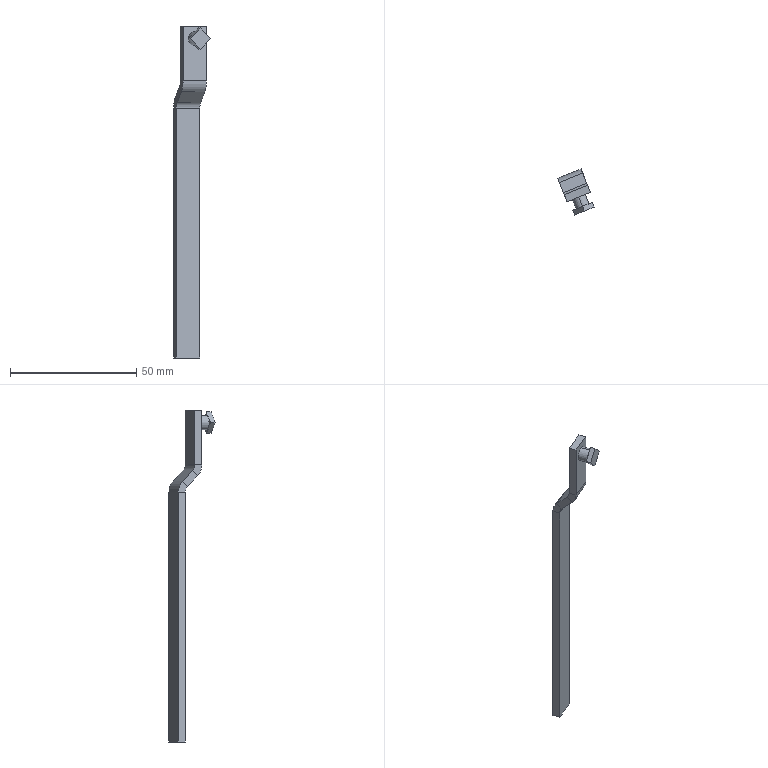Component | SolidWorks | RightDoorAssembly-1_LinkRodLock-1_Lock-1_UpperRod-1 | 1 solid | 30 faces | box 14.56 x 18.3 x 131.5 mm | volume 4187 mm3 | plane 24 | cylinder 6 | commonest cylinder face diameters 5.5 x2 6 x2 12 x2
STEP:
#1=COLOUR_RGB('',0.7922,0.8196,0.9333);
#2=FILL_AREA_STYLE_COLOUR('',#1);
#3=FILL_AREA_STYLE('',(#2));
#4=SURFACE_STYLE_FILL_AREA(#3);
#5=SURFACE_SIDE_STYLE('',(#4));
#6=SURFACE_STYLE_USAGE(.BOTH.,#5);
#7=PRESENTATION_STYLE_ASSIGNMENT((#6));
#8=CARTESIAN_POINT('',(-12.815,15.759,40.707));
#9=VERTEX_POINT('',#8);
#10=CARTESIAN_POINT('',(-12.815,15.759,40.49));
#11=VERTEX_POINT('',#10);
#12=CARTESIAN_POINT('',(-12.815,15.759,40.598));
#13=DIRECTION('',(0.3744,-0.9273,0.));
#14=DIRECTION('',(0.,0.,1.));
#15=AXIS2_PLACEMENT_3D('',#12,#13,#14);
#16=CIRCLE('',#15,0.1083);
#17=EDGE_CURVE('',#9,#11,#16,.T.);
#18=ORIENTED_EDGE('',*,*,#17,.F.);
#19=CARTESIAN_POINT('',(-12.874,15.905,40.707));
#20=VERTEX_POINT('',#19);
#21=CARTESIAN_POINT('',(-12.815,15.759,40.707));
#22=DIRECTION('',(-0.3744,0.9273,-0.));
#23=VECTOR('',#22,39.37);
#24=LINE('',#21,#23);
#25=EDGE_CURVE('',#9,#20,#24,.T.);
#26=ORIENTED_EDGE('',*,*,#25,.T.);
#27=CARTESIAN_POINT('',(-12.874,15.905,40.49));
#28=VERTEX_POINT('',#27);
#29=CARTESIAN_POINT('',(-12.874,15.905,40.598));
#30=DIRECTION('',(0.3744,-0.9273,0.));
#31=DIRECTION('',(0.,0.,-1.));
#32=AXIS2_PLACEMENT_3D('',#29,#30,#31);
#33=CIRCLE('',#32,0.1083);
#34=EDGE_CURVE('',#20,#28,#33,.T.);
#35=ORIENTED_EDGE('',*,*,#34,.T.);
#36=CARTESIAN_POINT('',(-12.815,15.759,40.49));
#37=DIRECTION('',(-0.3744,0.9273,-0.));
#38=VECTOR('',#37,39.37);
#39=LINE('',#36,#38);
#40=EDGE_CURVE('',#11,#28,#39,.T.);
#41=ORIENTED_EDGE('',*,*,#40,.F.);
#42=EDGE_LOOP('',(#18,#26,#35,#41));
#43=FACE_OUTER_BOUND('',#42,.T.);
#44=CARTESIAN_POINT('',(-12.815,15.759,40.598));
#45=DIRECTION('',(-0.3744,0.9273,-0.));
#46=DIRECTION('',(0.,0.,-1.));
#47=AXIS2_PLACEMENT_3D('',#44,#45,#46);
#48=CYLINDRICAL_SURFACE('',#47,0.1083);
#49=ADVANCED_FACE('',(#43),#48,.T.);
#50=CARTESIAN_POINT('',(-12.691,15.979,39.939));
#51=VERTEX_POINT('',#50);
#52=CARTESIAN_POINT('',(-12.691,15.979,40.795));
#53=VERTEX_POINT('',#52);
#54=CARTESIAN_POINT('',(-12.691,15.979,39.939));
#55=DIRECTION('',(-0.,0.,1.));
#56=VECTOR('',#55,39.37);
#57=LINE('',#54,#56);
#58=EDGE_CURVE('',#51,#53,#57,.T.);
#59=ORIENTED_EDGE('',*,*,#58,.T.);
#60=CARTESIAN_POINT('',(-13.056,15.832,40.795));
#61=VERTEX_POINT('',#60);
#62=CARTESIAN_POINT('',(-13.056,15.832,40.795));
#63=DIRECTION('',(0.9273,0.3744,0.));
#64=VECTOR('',#63,39.37);
#65=LINE('',#62,#64);
#66=EDGE_CURVE('',#61,#53,#65,.T.);
#67=ORIENTED_EDGE('',*,*,#66,.F.);
#68=CARTESIAN_POINT('',(-13.056,15.832,39.939));
#69=VERTEX_POINT('',#68);
#70=CARTESIAN_POINT('',(-13.056,15.832,39.939));
#71=DIRECTION('',(-0.,0.,1.));
#72=VECTOR('',#71,39.37);
#73=LINE('',#70,#72);
#74=EDGE_CURVE('',#69,#61,#73,.T.);
#75=ORIENTED_EDGE('',*,*,#74,.F.);
#76=CARTESIAN_POINT('',(-13.056,15.832,39.939));
#77=DIRECTION('',(0.9273,0.3744,0.));
#78=VECTOR('',#77,39.37);
#79=LINE('',#76,#78);
#80=EDGE_CURVE('',#69,#51,#79,.T.);
#81=ORIENTED_EDGE('',*,*,#80,.T.);
#82=EDGE_LOOP('',(#59,#67,#75,#81));
#83=FACE_OUTER_BOUND('',#82,.T.);
#84=CARTESIAN_POINT('',(-12.874,15.905,40.598));
#85=DIRECTION('',(0.3744,-0.9273,0.));
#86=DIRECTION('',(0.,0.,-1.));
#87=AXIS2_PLACEMENT_3D('',#84,#85,#86);
#88=CIRCLE('',#87,0.1083);
#89=EDGE_CURVE('',#28,#20,#88,.T.);
#90=ORIENTED_EDGE('',*,*,#89,.F.);
#91=ORIENTED_EDGE('',*,*,#34,.F.);
#92=EDGE_LOOP('',(#90,#91));
#93=FACE_BOUND('',#92,.T.);
#94=CARTESIAN_POINT('',(-13.056,15.832,39.939));
#95=DIRECTION('',(-0.3744,0.9273,-0.));
#96=DIRECTION('',(0.,-0.,-1.));
#97=AXIS2_PLACEMENT_3D('',#94,#95,#96);
#98=PLANE('',#97);
#99=ADVANCED_FACE('',(#83,#93),#98,.F.);
#100=CARTESIAN_POINT('',(-13.178,16.133,39.683));
#101=VERTEX_POINT('',#100);
#102=CARTESIAN_POINT('',(-13.146,16.055,39.6));
#103=VERTEX_POINT('',#102);
#104=CARTESIAN_POINT('',(-13.178,16.133,39.683));
#105=DIRECTION('',(0.2647,-0.6557,-0.7071));
#106=VECTOR('',#105,39.37);
#107=LINE('',#104,#106);
#108=EDGE_CURVE('',#101,#103,#107,.T.);
#109=ORIENTED_EDGE('',*,*,#108,.F.);
#110=CARTESIAN_POINT('',(-13.204,16.197,39.516));
#111=VERTEX_POINT('',#110);
#112=CARTESIAN_POINT('',(-13.115,15.978,39.516));
#113=DIRECTION('',(0.9273,0.3744,0.));
#114=DIRECTION('',(0.3744,-0.9273,0.));
#115=AXIS2_PLACEMENT_3D('',#112,#113,#114);
#116=CIRCLE('',#115,0.2362);
#117=EDGE_CURVE('',#111,#101,#116,.T.);
#118=ORIENTED_EDGE('',*,*,#117,.F.);
#119=CARTESIAN_POINT('',(-13.159,16.087,39.516));
#120=VERTEX_POINT('',#119);
#121=CARTESIAN_POINT('',(-13.159,16.087,39.516));
#122=DIRECTION('',(-0.3744,0.9273,-0.));
#123=VECTOR('',#122,39.37);
#124=LINE('',#121,#123);
#125=EDGE_CURVE('',#120,#111,#124,.T.);
#126=ORIENTED_EDGE('',*,*,#125,.F.);
#127=CARTESIAN_POINT('',(-13.115,15.978,39.516));
#128=DIRECTION('',(0.9273,0.3744,0.));
#129=DIRECTION('',(0.3744,-0.9273,-0.));
#130=AXIS2_PLACEMENT_3D('',#127,#128,#129);
#131=CIRCLE('',#130,0.1181);
#132=EDGE_CURVE('',#120,#103,#131,.T.);
#133=ORIENTED_EDGE('',*,*,#132,.T.);
#134=EDGE_LOOP('',(#109,#118,#126,#133));
#135=FACE_OUTER_BOUND('',#134,.T.);
#136=CARTESIAN_POINT('',(-13.178,16.133,39.683));
#137=DIRECTION('',(-0.9273,-0.3744,-0.));
#138=DIRECTION('',(0.3744,-0.9273,0.));
#139=AXIS2_PLACEMENT_3D('',#136,#137,#138);
#140=PLANE('',#139);
#141=ADVANCED_FACE('',(#135),#140,.T.);
#142=CARTESIAN_POINT('',(-13.113,15.973,39.855));
#143=VERTEX_POINT('',#142);
#144=CARTESIAN_POINT('',(-13.178,16.133,39.683));
#145=DIRECTION('',(0.2647,-0.6557,0.7071));
#146=VECTOR('',#145,39.37);
#147=LINE('',#144,#146);
#148=EDGE_CURVE('',#101,#143,#147,.T.);
#149=ORIENTED_EDGE('',*,*,#148,.F.);
#150=ORIENTED_EDGE('',*,*,#108,.T.);
#151=CARTESIAN_POINT('',(-13.082,15.896,39.772));
#152=VERTEX_POINT('',#151);
#153=CARTESIAN_POINT('',(-13.146,16.055,39.6));
#154=DIRECTION('',(0.2647,-0.6557,0.7071));
#155=VECTOR('',#154,39.37);
#156=LINE('',#153,#155);
#157=EDGE_CURVE('',#103,#152,#156,.T.);
#158=ORIENTED_EDGE('',*,*,#157,.T.);
#159=CARTESIAN_POINT('',(-13.082,15.896,39.772));
#160=DIRECTION('',(-0.2647,0.6557,0.7071));
#161=VECTOR('',#160,39.37);
#162=LINE('',#159,#161);
#163=EDGE_CURVE('',#152,#143,#162,.T.);
#164=ORIENTED_EDGE('',*,*,#163,.T.);
#165=EDGE_LOOP('',(#149,#150,#158,#164));
#166=FACE_OUTER_BOUND('',#165,.T.);
#167=CARTESIAN_POINT('',(-13.159,16.087,39.516));
#168=DIRECTION('',(-0.9273,-0.3744,-0.));
#169=DIRECTION('',(0.3744,-0.9273,0.));
#170=AXIS2_PLACEMENT_3D('',#167,#168,#169);
#171=PLANE('',#170);
#172=ADVANCED_FACE('',(#166),#171,.T.);
#173=CARTESIAN_POINT('',(-12.839,16.344,39.516));
#174=VERTEX_POINT('',#173);
#175=CARTESIAN_POINT('',(-12.794,16.235,39.516));
#176=VERTEX_POINT('',#175);
#177=CARTESIAN_POINT('',(-12.839,16.344,39.516));
#178=DIRECTION('',(0.3744,-0.9273,0.));
#179=VECTOR('',#178,39.37);
#180=LINE('',#177,#179);
#181=EDGE_CURVE('',#174,#176,#180,.T.);
#182=ORIENTED_EDGE('',*,*,#181,.F.);
#183=CARTESIAN_POINT('',(-12.813,16.28,39.683));
#184=VERTEX_POINT('',#183);
#185=CARTESIAN_POINT('',(-12.75,16.125,39.516));
#186=DIRECTION('',(0.9273,0.3744,0.));
#187=DIRECTION('',(0.3744,-0.9273,0.));
#188=AXIS2_PLACEMENT_3D('',#185,#186,#187);
#189=CIRCLE('',#188,0.2362);
#190=EDGE_CURVE('',#174,#184,#189,.T.);
#191=ORIENTED_EDGE('',*,*,#190,.T.);
#192=CARTESIAN_POINT('',(-12.781,16.203,39.6));
#193=VERTEX_POINT('',#192);
#194=CARTESIAN_POINT('',(-12.781,16.203,39.6));
#195=DIRECTION('',(-0.2647,0.6557,0.7071));
#196=VECTOR('',#195,39.37);
#197=LINE('',#194,#196);
#198=EDGE_CURVE('',#193,#184,#197,.T.);
#199=ORIENTED_EDGE('',*,*,#198,.F.);
#200=CARTESIAN_POINT('',(-12.75,16.125,39.516));
#201=DIRECTION('',(0.9273,0.3744,0.));
#202=DIRECTION('',(0.3744,-0.9273,-0.));
#203=AXIS2_PLACEMENT_3D('',#200,#201,#202);
#204=CIRCLE('',#203,0.1181);
#205=EDGE_CURVE('',#176,#193,#204,.T.);
#206=ORIENTED_EDGE('',*,*,#205,.F.);
#207=EDGE_LOOP('',(#182,#191,#199,#206));
#208=FACE_OUTER_BOUND('',#207,.T.);
#209=CARTESIAN_POINT('',(-12.839,16.344,39.516));
#210=DIRECTION('',(0.9273,0.3744,0.));
#211=DIRECTION('',(-0.3744,0.9273,-0.));
#212=AXIS2_PLACEMENT_3D('',#209,#210,#211);
#213=PLANE('',#212);
#214=ADVANCED_FACE('',(#208),#213,.T.);
#215=CARTESIAN_POINT('',(-12.839,16.344,35.618));
#216=VERTEX_POINT('',#215);
#217=CARTESIAN_POINT('',(-12.839,16.344,39.516));
#218=DIRECTION('',(-0.,0.,1.));
#219=VECTOR('',#218,39.37);
#220=LINE('',#217,#219);
#221=EDGE_CURVE('',#216,#174,#220,.T.);
#222=ORIENTED_EDGE('',*,*,#221,.T.);
#223=ORIENTED_EDGE('',*,*,#181,.T.);
#224=CARTESIAN_POINT('',(-12.794,16.235,35.618));
#225=VERTEX_POINT('',#224);
#226=CARTESIAN_POINT('',(-12.794,16.235,39.516));
#227=DIRECTION('',(-0.,0.,1.));
#228=VECTOR('',#227,39.37);
#229=LINE('',#226,#228);
#230=EDGE_CURVE('',#225,#176,#229,.T.);
#231=ORIENTED_EDGE('',*,*,#230,.F.);
#232=CARTESIAN_POINT('',(-12.794,16.235,35.618));
#233=DIRECTION('',(-0.3744,0.9273,-0.));
#234=VECTOR('',#233,39.37);
#235=LINE('',#232,#234);
#236=EDGE_CURVE('',#225,#216,#235,.T.);
#237=ORIENTED_EDGE('',*,*,#236,.T.);
#238=EDGE_LOOP('',(#222,#223,#231,#237));
#239=FACE_OUTER_BOUND('',#238,.T.);
#240=CARTESIAN_POINT('',(-12.781,16.203,39.6));
#241=DIRECTION('',(0.9273,0.3744,0.));
#242=DIRECTION('',(-0.3744,0.9273,-0.));
#243=AXIS2_PLACEMENT_3D('',#240,#241,#242);
#244=PLANE('',#243);
#245=ADVANCED_FACE('',(#239),#244,.T.);
#246=CARTESIAN_POINT('',(-13.1,15.941,39.939));
#247=VERTEX_POINT('',#246);
#248=CARTESIAN_POINT('',(-13.1,15.941,39.939));
#249=DIRECTION('',(0.3744,-0.9273,0.));
#250=VECTOR('',#249,39.37);
#251=LINE('',#248,#250);
#252=EDGE_CURVE('',#247,#69,#251,.T.);
#253=ORIENTED_EDGE('',*,*,#252,.F.);
#254=CARTESIAN_POINT('',(-13.145,16.051,39.939));
#255=DIRECTION('',(-0.9273,-0.3744,-0.));
#256=DIRECTION('',(0.3744,-0.9273,0.));
#257=AXIS2_PLACEMENT_3D('',#254,#255,#256);
#258=CIRCLE('',#257,0.1181);
#259=EDGE_CURVE('',#143,#247,#258,.T.);
#260=ORIENTED_EDGE('',*,*,#259,.F.);
#261=ORIENTED_EDGE('',*,*,#163,.F.);
#262=CARTESIAN_POINT('',(-13.145,16.051,39.939));
#263=DIRECTION('',(-0.9273,-0.3744,-0.));
#264=DIRECTION('',(0.3744,-0.9273,0.));
#265=AXIS2_PLACEMENT_3D('',#262,#263,#264);
#266=CIRCLE('',#265,0.2362);
#267=EDGE_CURVE('',#152,#69,#266,.T.);
#268=ORIENTED_EDGE('',*,*,#267,.T.);
#269=EDGE_LOOP('',(#253,#260,#261,#268));
#270=FACE_OUTER_BOUND('',#269,.T.);
#271=CARTESIAN_POINT('',(-13.1,15.941,39.939));
#272=DIRECTION('',(-0.9273,-0.3744,-0.));
#273=DIRECTION('',(0.3744,-0.9273,0.));
#274=AXIS2_PLACEMENT_3D('',#271,#272,#273);
#275=PLANE('',#274);
#276=ADVANCED_FACE('',(#270),#275,.T.);
#277=CARTESIAN_POINT('',(-13.1,15.941,40.795));
#278=VERTEX_POINT('',#277);
#279=CARTESIAN_POINT('',(-13.1,15.941,39.939));
#280=DIRECTION('',(-0.,0.,1.));
#281=VECTOR('',#280,39.37);
#282=LINE('',#279,#281);
#283=EDGE_CURVE('',#247,#278,#282,.T.);
#284=ORIENTED_EDGE('',*,*,#283,.F.);
#285=ORIENTED_EDGE('',*,*,#252,.T.);
#286=ORIENTED_EDGE('',*,*,#74,.T.);
#287=CARTESIAN_POINT('',(-13.1,15.941,40.795));
#288=DIRECTION('',(0.3744,-0.9273,0.));
#289=VECTOR('',#288,39.37);
#290=LINE('',#287,#289);
#291=EDGE_CURVE('',#278,#61,#290,.T.);
#292=ORIENTED_EDGE('',*,*,#291,.F.);
#293=EDGE_LOOP('',(#284,#285,#286,#292));
#294=FACE_OUTER_BOUND('',#293,.T.);
#295=CARTESIAN_POINT('',(-13.082,15.896,39.772));
#296=DIRECTION('',(-0.9273,-0.3744,-0.));
#297=DIRECTION('',(0.3744,-0.9273,0.));
#298=AXIS2_PLACEMENT_3D('',#295,#296,#297);
#299=PLANE('',#298);
#300=ADVANCED_FACE('',(#294),#299,.T.);
#301=CARTESIAN_POINT('',(-12.748,16.121,39.855));
#302=VERTEX_POINT('',#301);
#303=CARTESIAN_POINT('',(-12.717,16.043,39.772));
#304=VERTEX_POINT('',#303);
#305=CARTESIAN_POINT('',(-12.748,16.121,39.855));
#306=DIRECTION('',(0.2647,-0.6557,-0.7071));
#307=VECTOR('',#306,39.37);
#308=LINE('',#305,#307);
#309=EDGE_CURVE('',#302,#304,#308,.T.);
#310=ORIENTED_EDGE('',*,*,#309,.F.);
#311=CARTESIAN_POINT('',(-12.735,16.089,39.939));
#312=VERTEX_POINT('',#311);
#313=CARTESIAN_POINT('',(-12.78,16.198,39.939));
#314=DIRECTION('',(-0.9273,-0.3744,-0.));
#315=DIRECTION('',(0.3744,-0.9273,0.));
#316=AXIS2_PLACEMENT_3D('',#313,#314,#315);
#317=CIRCLE('',#316,0.1181);
#318=EDGE_CURVE('',#302,#312,#317,.T.);
#319=ORIENTED_EDGE('',*,*,#318,.T.);
#320=CARTESIAN_POINT('',(-12.691,15.979,39.939));
#321=DIRECTION('',(-0.3744,0.9273,-0.));
#322=VECTOR('',#321,39.37);
#323=LINE('',#320,#322);
#324=EDGE_CURVE('',#51,#312,#323,.T.);
#325=ORIENTED_EDGE('',*,*,#324,.F.);
#326=CARTESIAN_POINT('',(-12.78,16.198,39.939));
#327=DIRECTION('',(-0.9273,-0.3744,-0.));
#328=DIRECTION('',(0.3744,-0.9273,0.));
#329=AXIS2_PLACEMENT_3D('',#326,#327,#328);
#330=CIRCLE('',#329,0.2362);
#331=EDGE_CURVE('',#304,#51,#330,.T.);
#332=ORIENTED_EDGE('',*,*,#331,.F.);
#333=EDGE_LOOP('',(#310,#319,#325,#332));
#334=FACE_OUTER_BOUND('',#333,.T.);
#335=CARTESIAN_POINT('',(-12.748,16.121,39.855));
#336=DIRECTION('',(0.9273,0.3744,0.));
#337=DIRECTION('',(-0.3744,0.9273,-0.));
#338=AXIS2_PLACEMENT_3D('',#335,#336,#337);
#339=PLANE('',#338);
#340=ADVANCED_FACE('',(#334),#339,.T.);
#341=CARTESIAN_POINT('',(-12.813,16.28,39.683));
#342=DIRECTION('',(0.2647,-0.6557,0.7071));
#343=VECTOR('',#342,39.37);
#344=LINE('',#341,#343);
#345=EDGE_CURVE('',#184,#302,#344,.T.);
#346=ORIENTED_EDGE('',*,*,#345,.T.);
#347=ORIENTED_EDGE('',*,*,#309,.T.);
#348=CARTESIAN_POINT('',(-12.781,16.203,39.6));
#349=DIRECTION('',(0.2647,-0.6557,0.7071));
#350=VECTOR('',#349,39.37);
#351=LINE('',#348,#350);
#352=EDGE_CURVE('',#193,#304,#351,.T.);
#353=ORIENTED_EDGE('',*,*,#352,.F.);
#354=ORIENTED_EDGE('',*,*,#198,.T.);
#355=EDGE_LOOP('',(#346,#347,#353,#354));
#356=FACE_OUTER_BOUND('',#355,.T.);
#357=CARTESIAN_POINT('',(-12.691,15.979,39.939));
#358=DIRECTION('',(0.9273,0.3744,0.));
#359=DIRECTION('',(-0.3744,0.9273,-0.));
#360=AXIS2_PLACEMENT_3D('',#357,#358,#359);
#361=PLANE('',#360);
#362=ADVANCED_FACE('',(#356),#361,.T.);
#363=CARTESIAN_POINT('',(-12.735,16.089,40.795));
#364=VERTEX_POINT('',#363);
#365=CARTESIAN_POINT('',(-12.735,16.089,40.795));
#366=DIRECTION('',(0.3744,-0.9273,0.));
#367=VECTOR('',#366,39.37);
#368=LINE('',#365,#367);
#369=EDGE_CURVE('',#364,#53,#368,.T.);
#370=ORIENTED_EDGE('',*,*,#369,.F.);
#371=CARTESIAN_POINT('',(-13.1,15.941,40.795));
#372=DIRECTION('',(0.9273,0.3744,0.));
#373=VECTOR('',#372,39.37);
#374=LINE('',#371,#373);
#375=EDGE_CURVE('',#278,#364,#374,.T.);
#376=ORIENTED_EDGE('',*,*,#375,.F.);
#377=ORIENTED_EDGE('',*,*,#291,.T.);
#378=ORIENTED_EDGE('',*,*,#66,.T.);
#379=EDGE_LOOP('',(#370,#376,#377,#378));
#380=FACE_OUTER_BOUND('',#379,.T.);
#381=CARTESIAN_POINT('',(-13.1,15.941,40.795));
#382=DIRECTION('',(-0.,0.,1.));
#383=DIRECTION('',(-0.3744,0.9273,-0.));
#384=AXIS2_PLACEMENT_3D('',#381,#382,#383);
#385=PLANE('',#384);
#386=ADVANCED_FACE('',(#380),#385,.T.);
#387=CARTESIAN_POINT('',(-12.735,16.089,39.939));
#388=DIRECTION('',(-0.,0.,1.));
#389=VECTOR('',#388,39.37);
#390=LINE('',#387,#389);
#391=EDGE_CURVE('',#312,#364,#390,.T.);
#392=ORIENTED_EDGE('',*,*,#391,.F.);
#393=CARTESIAN_POINT('',(-13.1,15.941,39.939));
#394=DIRECTION('',(0.9273,0.3744,0.));
#395=VECTOR('',#394,39.37);
#396=LINE('',#393,#395);
#397=EDGE_CURVE('',#247,#312,#396,.T.);
#398=ORIENTED_EDGE('',*,*,#397,.F.);
#399=ORIENTED_EDGE('',*,*,#283,.T.);
#400=ORIENTED_EDGE('',*,*,#375,.T.);
#401=EDGE_LOOP('',(#392,#398,#399,#400));
#402=FACE_OUTER_BOUND('',#401,.T.);
#403=CARTESIAN_POINT('',(-13.1,15.941,39.939));
#404=DIRECTION('',(-0.3744,0.9273,-0.));
#405=DIRECTION('',(0.,-0.,-1.));
#406=AXIS2_PLACEMENT_3D('',#403,#404,#405);
#407=PLANE('',#406);
#408=ADVANCED_FACE('',(#402),#407,.T.);
#409=ORIENTED_EDGE('',*,*,#318,.F.);
#410=CARTESIAN_POINT('',(-13.113,15.973,39.855));
#411=DIRECTION('',(0.9273,0.3744,0.));
#412=VECTOR('',#411,39.37);
#413=LINE('',#410,#412);
#414=EDGE_CURVE('',#143,#302,#413,.T.);
#415=ORIENTED_EDGE('',*,*,#414,.F.);
#416=ORIENTED_EDGE('',*,*,#259,.T.);
#417=ORIENTED_EDGE('',*,*,#397,.T.);
#418=EDGE_LOOP('',(#409,#415,#416,#417));
#419=FACE_OUTER_BOUND('',#418,.T.);
#420=CARTESIAN_POINT('',(-13.145,16.051,39.939));
#421=DIRECTION('',(0.9273,0.3744,0.));
#422=DIRECTION('',(-0.3744,0.9273,0.));
#423=AXIS2_PLACEMENT_3D('',#420,#421,#422);
#424=CYLINDRICAL_SURFACE('',#423,0.1181);
#425=ADVANCED_FACE('',(#419),#424,.F.);
#426=ORIENTED_EDGE('',*,*,#345,.F.);
#427=CARTESIAN_POINT('',(-13.178,16.133,39.683));
#428=DIRECTION('',(0.9273,0.3744,0.));
#429=VECTOR('',#428,39.37);
#430=LINE('',#427,#429);
#431=EDGE_CURVE('',#101,#184,#430,.T.);
#432=ORIENTED_EDGE('',*,*,#431,.F.);
#433=ORIENTED_EDGE('',*,*,#148,.T.);
#434=ORIENTED_EDGE('',*,*,#414,.T.);
#435=EDGE_LOOP('',(#426,#432,#433,#434));
#436=FACE_OUTER_BOUND('',#435,.T.);
#437=CARTESIAN_POINT('',(-13.178,16.133,39.683));
#438=DIRECTION('',(-0.2647,0.6557,0.7071));
#439=DIRECTION('',(-0.2647,0.6557,-0.7071));
#440=AXIS2_PLACEMENT_3D('',#437,#438,#439);
#441=PLANE('',#440);
#442=ADVANCED_FACE('',(#436),#441,.T.);
#443=ORIENTED_EDGE('',*,*,#190,.F.);
#444=CARTESIAN_POINT('',(-13.204,16.197,39.516));
#445=DIRECTION('',(0.9273,0.3744,0.));
#446=VECTOR('',#445,39.37);
#447=LINE('',#444,#446);
#448=EDGE_CURVE('',#111,#174,#447,.T.);
#449=ORIENTED_EDGE('',*,*,#448,.F.);
#450=ORIENTED_EDGE('',*,*,#117,.T.);
#451=ORIENTED_EDGE('',*,*,#431,.T.);
#452=EDGE_LOOP('',(#443,#449,#450,#451));
#453=FACE_OUTER_BOUND('',#452,.T.);
#454=CARTESIAN_POINT('',(-13.115,15.978,39.516));
#455=DIRECTION('',(0.9273,0.3744,0.));
#456=DIRECTION('',(-0.3744,0.9273,0.));
#457=AXIS2_PLACEMENT_3D('',#454,#455,#456);
#458=CYLINDRICAL_SURFACE('',#457,0.2362);
#459=ADVANCED_FACE('',(#453),#458,.T.);
#460=ORIENTED_EDGE('',*,*,#221,.F.);
#461=CARTESIAN_POINT('',(-13.204,16.197,35.618));
#462=VERTEX_POINT('',#461);
#463=CARTESIAN_POINT('',(-13.204,16.197,35.618));
#464=DIRECTION('',(0.9273,0.3744,0.));
#465=VECTOR('',#464,39.37);
#466=LINE('',#463,#465);
#467=EDGE_CURVE('',#462,#216,#466,.T.);
#468=ORIENTED_EDGE('',*,*,#467,.F.);
#469=CARTESIAN_POINT('',(-13.204,16.197,39.516));
#470=DIRECTION('',(-0.,0.,1.));
#471=VECTOR('',#470,39.37);
#472=LINE('',#469,#471);
#473=EDGE_CURVE('',#462,#111,#472,.T.);
#474=ORIENTED_EDGE('',*,*,#473,.T.);
#475=ORIENTED_EDGE('',*,*,#448,.T.);
#476=EDGE_LOOP('',(#460,#468,#474,#475));
#477=FACE_OUTER_BOUND('',#476,.T.);
#478=CARTESIAN_POINT('',(-13.204,16.197,39.516));
#479=DIRECTION('',(-0.3744,0.9273,-0.));
#480=DIRECTION('',(-0.9273,-0.3744,-0.));
#481=AXIS2_PLACEMENT_3D('',#478,#479,#480);
#482=PLANE('',#481);
#483=ADVANCED_FACE('',(#477),#482,.T.);
#484=ORIENTED_EDGE('',*,*,#236,.F.);
#485=CARTESIAN_POINT('',(-13.159,16.087,35.618));
#486=VERTEX_POINT('',#485);
#487=CARTESIAN_POINT('',(-13.159,16.087,35.618));
#488=DIRECTION('',(0.9273,0.3744,0.));
#489=VECTOR('',#488,39.37);
#490=LINE('',#487,#489);
#491=EDGE_CURVE('',#486,#225,#490,.T.);
#492=ORIENTED_EDGE('',*,*,#491,.F.);
#493=CARTESIAN_POINT('',(-13.159,16.087,35.618));
#494=DIRECTION('',(-0.3744,0.9273,-0.));
#495=VECTOR('',#494,39.37);
#496=LINE('',#493,#495);
#497=EDGE_CURVE('',#486,#462,#496,.T.);
#498=ORIENTED_EDGE('',*,*,#497,.T.);
#499=ORIENTED_EDGE('',*,*,#467,.T.);
#500=EDGE_LOOP('',(#484,#492,#498,#499));
#501=FACE_OUTER_BOUND('',#500,.T.);
#502=CARTESIAN_POINT('',(-13.159,16.087,35.618));
#503=DIRECTION('',(0.,-0.,-1.));
#504=DIRECTION('',(0.9273,0.3744,0.));
#505=AXIS2_PLACEMENT_3D('',#502,#503,#504);
#506=PLANE('',#505);
#507=ADVANCED_FACE('',(#501),#506,.T.);
#508=ORIENTED_EDGE('',*,*,#230,.T.);
#509=CARTESIAN_POINT('',(-13.159,16.087,39.516));
#510=DIRECTION('',(0.9273,0.3744,0.));
#511=VECTOR('',#510,39.37);
#512=LINE('',#509,#511);
#513=EDGE_CURVE('',#120,#176,#512,.T.);
#514=ORIENTED_EDGE('',*,*,#513,.F.);
#515=CARTESIAN_POINT('',(-13.159,16.087,39.516));
#516=DIRECTION('',(-0.,0.,1.));
#517=VECTOR('',#516,39.37);
#518=LINE('',#515,#517);
#519=EDGE_CURVE('',#486,#120,#518,.T.);
#520=ORIENTED_EDGE('',*,*,#519,.F.);
#521=ORIENTED_EDGE('',*,*,#491,.T.);
#522=EDGE_LOOP('',(#508,#514,#520,#521));
#523=FACE_OUTER_BOUND('',#522,.T.);
#524=CARTESIAN_POINT('',(-13.159,16.087,39.516));
#525=DIRECTION('',(-0.3744,0.9273,-0.));
#526=DIRECTION('',(-0.9273,-0.3744,-0.));
#527=AXIS2_PLACEMENT_3D('',#524,#525,#526);
#528=PLANE('',#527);
#529=ADVANCED_FACE('',(#523),#528,.F.);
#530=ORIENTED_EDGE('',*,*,#205,.T.);
#531=CARTESIAN_POINT('',(-13.146,16.055,39.6));
#532=DIRECTION('',(0.9273,0.3744,0.));
#533=VECTOR('',#532,39.37);
#534=LINE('',#531,#533);
#535=EDGE_CURVE('',#103,#193,#534,.T.);
#536=ORIENTED_EDGE('',*,*,#535,.F.);
#537=ORIENTED_EDGE('',*,*,#132,.F.);
#538=ORIENTED_EDGE('',*,*,#513,.T.);
#539=EDGE_LOOP('',(#530,#536,#537,#538));
#540=FACE_OUTER_BOUND('',#539,.T.);
#541=CARTESIAN_POINT('',(-13.115,15.978,39.516));
#542=DIRECTION('',(0.9273,0.3744,0.));
#543=DIRECTION('',(-0.3744,0.9273,0.));
#544=AXIS2_PLACEMENT_3D('',#541,#542,#543);
#545=CYLINDRICAL_SURFACE('',#544,0.1181);
#546=ADVANCED_FACE('',(#540),#545,.F.);
#547=ORIENTED_EDGE('',*,*,#352,.T.);
#548=CARTESIAN_POINT('',(-13.082,15.896,39.772));
#549=DIRECTION('',(0.9273,0.3744,0.));
#550=VECTOR('',#549,39.37);
#551=LINE('',#548,#550);
#552=EDGE_CURVE('',#152,#304,#551,.T.);
#553=ORIENTED_EDGE('',*,*,#552,.F.);
#554=ORIENTED_EDGE('',*,*,#157,.F.);
#555=ORIENTED_EDGE('',*,*,#535,.T.);
#556=EDGE_LOOP('',(#547,#553,#554,#555));
#557=FACE_OUTER_BOUND('',#556,.T.);
#558=CARTESIAN_POINT('',(-13.146,16.055,39.6));
#559=DIRECTION('',(-0.2647,0.6557,0.7071));
#560=DIRECTION('',(-0.2647,0.6557,-0.7071));
#561=AXIS2_PLACEMENT_3D('',#558,#559,#560);
#562=PLANE('',#561);
#563=ADVANCED_FACE('',(#557),#562,.F.);
#564=ORIENTED_EDGE('',*,*,#331,.T.);
#565=ORIENTED_EDGE('',*,*,#80,.F.);
#566=ORIENTED_EDGE('',*,*,#267,.F.);
#567=ORIENTED_EDGE('',*,*,#552,.T.);
#568=EDGE_LOOP('',(#564,#565,#566,#567));
#569=FACE_OUTER_BOUND('',#568,.T.);
#570=CARTESIAN_POINT('',(-13.145,16.051,39.939));
#571=DIRECTION('',(0.9273,0.3744,0.));
#572=DIRECTION('',(-0.3744,0.9273,0.));
#573=AXIS2_PLACEMENT_3D('',#570,#571,#572);
#574=CYLINDRICAL_SURFACE('',#573,0.2362);
#575=ADVANCED_FACE('',(#569),#574,.T.);
#576=ORIENTED_EDGE('',*,*,#519,.T.);
#577=ORIENTED_EDGE('',*,*,#125,.T.);
#578=ORIENTED_EDGE('',*,*,#473,.F.);
#579=ORIENTED_EDGE('',*,*,#497,.F.);
#580=EDGE_LOOP('',(#576,#577,#578,#579));
#581=FACE_OUTER_BOUND('',#580,.T.);
#582=CARTESIAN_POINT('',(-13.145,16.051,39.939));
#583=DIRECTION('',(-0.9273,-0.3744,-0.));
#584=DIRECTION('',(0.3744,-0.9273,0.));
#585=AXIS2_PLACEMENT_3D('',#582,#583,#584);
#586=PLANE('',#585);
#587=ADVANCED_FACE('',(#581),#586,.T.);
#588=ORIENTED_EDGE('',*,*,#58,.F.);
#589=ORIENTED_EDGE('',*,*,#324,.T.);
#590=ORIENTED_EDGE('',*,*,#391,.T.);
#591=ORIENTED_EDGE('',*,*,#369,.T.);
#592=EDGE_LOOP('',(#588,#589,#590,#591));
#593=FACE_OUTER_BOUND('',#592,.T.);
#594=CARTESIAN_POINT('',(-12.78,16.198,39.939));
#595=DIRECTION('',(-0.9273,-0.3744,-0.));
#596=DIRECTION('',(0.3744,-0.9273,0.));
#597=AXIS2_PLACEMENT_3D('',#594,#595,#596);
#598=PLANE('',#597);
#599=ADVANCED_FACE('',(#593),#598,.F.);
#600=ORIENTED_EDGE('',*,*,#25,.F.);
#601=CARTESIAN_POINT('',(-12.815,15.759,40.598));
#602=DIRECTION('',(0.3744,-0.9273,0.));
#603=DIRECTION('',(0.,0.,1.));
#604=AXIS2_PLACEMENT_3D('',#601,#602,#603);
#605=CIRCLE('',#604,0.1083);
#606=EDGE_CURVE('',#11,#9,#605,.T.);
#607=ORIENTED_EDGE('',*,*,#606,.F.);
#608=ORIENTED_EDGE('',*,*,#40,.T.);
#609=ORIENTED_EDGE('',*,*,#89,.T.);
#610=EDGE_LOOP('',(#600,#607,#608,#609));
#611=FACE_OUTER_BOUND('',#610,.T.);
#612=CARTESIAN_POINT('',(-12.815,15.759,40.598));
#613=DIRECTION('',(-0.3744,0.9273,-0.));
#614=DIRECTION('',(0.,0.,-1.));
#615=AXIS2_PLACEMENT_3D('',#612,#613,#614);
#616=CYLINDRICAL_SURFACE('',#615,0.1083);
#617=ADVANCED_FACE('',(#611),#616,.T.);
#618=CARTESIAN_POINT('',(-12.815,15.759,40.765));
#619=VERTEX_POINT('',#618);
#620=CARTESIAN_POINT('',(-12.97,15.697,40.598));
#621=VERTEX_POINT('',#620);
#622=CARTESIAN_POINT('',(-12.815,15.759,40.765));
#623=DIRECTION('',(-0.6557,-0.2647,-0.7071));
#624=VECTOR('',#623,39.37);
#625=LINE('',#622,#624);
#626=EDGE_CURVE('',#619,#621,#625,.T.);
#627=ORIENTED_EDGE('',*,*,#626,.F.);
#628=CARTESIAN_POINT('',(-12.66,15.822,40.598));
#629=VERTEX_POINT('',#628);
#630=CARTESIAN_POINT('',(-12.815,15.759,40.765));
#631=DIRECTION('',(-0.6557,-0.2647,0.7071));
#632=VECTOR('',#631,39.37);
#633=LINE('',#630,#632);
#634=EDGE_CURVE('',#629,#619,#633,.T.);
#635=ORIENTED_EDGE('',*,*,#634,.F.);
#636=CARTESIAN_POINT('',(-12.815,15.759,40.431));
#637=VERTEX_POINT('',#636);
#638=CARTESIAN_POINT('',(-12.66,15.822,40.598));
#639=DIRECTION('',(0.6557,0.2647,0.7071));
#640=VECTOR('',#639,39.37);
#641=LINE('',#638,#640);
#642=EDGE_CURVE('',#637,#629,#641,.T.);
#643=ORIENTED_EDGE('',*,*,#642,.F.);
#644=CARTESIAN_POINT('',(-12.97,15.697,40.598));
#645=DIRECTION('',(0.6557,0.2647,-0.7071));
#646=VECTOR('',#645,39.37);
#647=LINE('',#644,#646);
#648=EDGE_CURVE('',#621,#637,#647,.T.);
#649=ORIENTED_EDGE('',*,*,#648,.F.);
#650=EDGE_LOOP('',(#627,#635,#643,#649));
#651=FACE_OUTER_BOUND('',#650,.T.);
#652=ORIENTED_EDGE('',*,*,#606,.T.);
#653=ORIENTED_EDGE('',*,*,#17,.T.);
#654=EDGE_LOOP('',(#652,#653));
#655=FACE_BOUND('',#654,.T.);
#656=CARTESIAN_POINT('',(-12.97,15.697,40.598));
#657=DIRECTION('',(0.3744,-0.9273,0.));
#658=DIRECTION('',(-0.,0.,1.));
#659=AXIS2_PLACEMENT_3D('',#656,#657,#658);
#660=PLANE('',#659);
#661=ADVANCED_FACE('',(#651,#655),#660,.F.);
#662=ORIENTED_EDGE('',*,*,#626,.T.);
#663=CARTESIAN_POINT('',(-12.94,15.624,40.598));
#664=VERTEX_POINT('',#663);
#665=CARTESIAN_POINT('',(-12.94,15.624,40.598));
#666=DIRECTION('',(-0.3744,0.9273,-0.));
#667=VECTOR('',#666,39.37);
#668=LINE('',#665,#667);
#669=EDGE_CURVE('',#664,#621,#668,.T.);
#670=ORIENTED_EDGE('',*,*,#669,.F.);
#671=CARTESIAN_POINT('',(-12.785,15.686,40.765));
#672=VERTEX_POINT('',#671);
#673=CARTESIAN_POINT('',(-12.785,15.686,40.765));
#674=DIRECTION('',(-0.6557,-0.2647,-0.7071));
#675=VECTOR('',#674,39.37);
#676=LINE('',#673,#675);
#677=EDGE_CURVE('',#672,#664,#676,.T.);
#678=ORIENTED_EDGE('',*,*,#677,.F.);
#679=CARTESIAN_POINT('',(-12.785,15.686,40.765));
#680=DIRECTION('',(-0.3744,0.9273,-0.));
#681=VECTOR('',#680,39.37);
#682=LINE('',#679,#681);
#683=EDGE_CURVE('',#672,#619,#682,.T.);
#684=ORIENTED_EDGE('',*,*,#683,.T.);
#685=EDGE_LOOP('',(#662,#670,#678,#684));
#686=FACE_OUTER_BOUND('',#685,.T.);
#687=CARTESIAN_POINT('',(-12.785,15.686,40.765));
#688=DIRECTION('',(0.6557,0.2647,-0.7071));
#689=DIRECTION('',(0.6557,0.2647,0.7071));
#690=AXIS2_PLACEMENT_3D('',#687,#688,#689);
#691=PLANE('',#690);
#692=ADVANCED_FACE('',(#686),#691,.F.);
#693=ORIENTED_EDGE('',*,*,#648,.T.);
#694=CARTESIAN_POINT('',(-12.785,15.686,40.431));
#695=VERTEX_POINT('',#694);
#696=CARTESIAN_POINT('',(-12.785,15.686,40.431));
#697=DIRECTION('',(-0.3744,0.9273,-0.));
#698=VECTOR('',#697,39.37);
#699=LINE('',#696,#698);
#700=EDGE_CURVE('',#695,#637,#699,.T.);
#701=ORIENTED_EDGE('',*,*,#700,.F.);
#702=CARTESIAN_POINT('',(-12.94,15.624,40.598));
#703=DIRECTION('',(0.6557,0.2647,-0.7071));
#704=VECTOR('',#703,39.37);
#705=LINE('',#702,#704);
#706=EDGE_CURVE('',#664,#695,#705,.T.);
#707=ORIENTED_EDGE('',*,*,#706,.F.);
#708=ORIENTED_EDGE('',*,*,#669,.T.);
#709=EDGE_LOOP('',(#693,#701,#707,#708));
#710=FACE_OUTER_BOUND('',#709,.T.);
#711=CARTESIAN_POINT('',(-12.94,15.624,40.598));
#712=DIRECTION('',(0.6557,0.2647,0.7071));
#713=DIRECTION('',(-0.6557,-0.2647,0.7071));
#714=AXIS2_PLACEMENT_3D('',#711,#712,#713);
#715=PLANE('',#714);
#716=ADVANCED_FACE('',(#710),#715,.F.);
#717=ORIENTED_EDGE('',*,*,#642,.T.);
#718=CARTESIAN_POINT('',(-12.63,15.749,40.598));
#719=VERTEX_POINT('',#718);
#720=CARTESIAN_POINT('',(-12.63,15.749,40.598));
#721=DIRECTION('',(-0.3744,0.9273,-0.));
#722=VECTOR('',#721,39.37);
#723=LINE('',#720,#722);
#724=EDGE_CURVE('',#719,#629,#723,.T.);
#725=ORIENTED_EDGE('',*,*,#724,.F.);
#726=CARTESIAN_POINT('',(-12.63,15.749,40.598));
#727=DIRECTION('',(0.6557,0.2647,0.7071));
#728=VECTOR('',#727,39.37);
#729=LINE('',#726,#728);
#730=EDGE_CURVE('',#695,#719,#729,.T.);
#731=ORIENTED_EDGE('',*,*,#730,.F.);
#732=ORIENTED_EDGE('',*,*,#700,.T.);
#733=EDGE_LOOP('',(#717,#725,#731,#732));
#734=FACE_OUTER_BOUND('',#733,.T.);
#735=CARTESIAN_POINT('',(-12.63,15.749,40.598));
#736=DIRECTION('',(-0.6557,-0.2647,0.7071));
#737=DIRECTION('',(-0.6557,-0.2647,-0.7071));
#738=AXIS2_PLACEMENT_3D('',#735,#736,#737);
#739=PLANE('',#738);
#740=ADVANCED_FACE('',(#734),#739,.F.);
#741=ORIENTED_EDGE('',*,*,#634,.T.);
#742=ORIENTED_EDGE('',*,*,#683,.F.);
#743=CARTESIAN_POINT('',(-12.785,15.686,40.765));
#744=DIRECTION('',(-0.6557,-0.2647,0.7071));
#745=VECTOR('',#744,39.37);
#746=LINE('',#743,#745);
#747=EDGE_CURVE('',#719,#672,#746,.T.);
#748=ORIENTED_EDGE('',*,*,#747,.F.);
#749=ORIENTED_EDGE('',*,*,#724,.T.);
#750=EDGE_LOOP('',(#741,#742,#748,#749));
#751=FACE_OUTER_BOUND('',#750,.T.);
#752=CARTESIAN_POINT('',(-12.785,15.686,40.765));
#753=DIRECTION('',(-0.6557,-0.2647,-0.7071));
#754=DIRECTION('',(0.6557,0.2647,-0.7071));
#755=AXIS2_PLACEMENT_3D('',#752,#753,#754);
#756=PLANE('',#755);
#757=ADVANCED_FACE('',(#751),#756,.F.);
#758=ORIENTED_EDGE('',*,*,#677,.T.);
#759=ORIENTED_EDGE('',*,*,#706,.T.);
#760=ORIENTED_EDGE('',*,*,#730,.T.);
#761=ORIENTED_EDGE('',*,*,#747,.T.);
#762=EDGE_LOOP('',(#758,#759,#760,#761));
#763=FACE_OUTER_BOUND('',#762,.T.);
#764=CARTESIAN_POINT('',(-12.94,15.624,40.598));
#765=DIRECTION('',(0.3744,-0.9273,0.));
#766=DIRECTION('',(-0.,0.,1.));
#767=AXIS2_PLACEMENT_3D('',#764,#765,#766);
#768=PLANE('',#767);
#769=ADVANCED_FACE('',(#763),#768,.T.);
#770=CLOSED_SHELL('',(#49,#99,#141,#172,#214,#245,#276,#300,#340,#362,#386,#408,#425,#442,#459,#483,#507,#529,#546,#563,#575,#587,#599,#617,#661,#692,#716,#740,#757,#769));
#771=MANIFOLD_SOLID_BREP('',#770);
#772=STYLED_ITEM('',(#7),#771);
#773=PRESENTATION_LAYER_ASSIGNMENT('','',(#772));
#774=CARTESIAN_POINT('',(0.,0.,0.));
#775=DIRECTION('',(0.,0.,1.));
#776=DIRECTION('',(1.,0.,0.));
#777=AXIS2_PLACEMENT_3D('',#774,#775,#776);
#778=(LENGTH_UNIT()NAMED_UNIT(*)SI_UNIT($,.METRE.));
#779=LENGTH_MEASURE_WITH_UNIT(LENGTH_MEASURE(0.0254),#778);
#780=DIMENSIONAL_EXPONENTS(1.,0.,0.,0.,0.,0.,0.);
#781=(CONVERSION_BASED_UNIT('',#779)LENGTH_UNIT()NAMED_UNIT(#780));
#782=UNCERTAINTY_MEASURE_WITH_UNIT(LENGTH_MEASURE(0.00001),#781,'','');
#783=(NAMED_UNIT(*)PLANE_ANGLE_UNIT()SI_UNIT($,.RADIAN.));
#784=(NAMED_UNIT(*)SI_UNIT($,.STERADIAN.)SOLID_ANGLE_UNIT());
#785=(GEOMETRIC_REPRESENTATION_CONTEXT(3)GLOBAL_UNCERTAINTY_ASSIGNED_CONTEXT((#782))GLOBAL_UNIT_ASSIGNED_CONTEXT((#781,#783,#784))REPRESENTATION_CONTEXT('',''));
#786=ADVANCED_BREP_SHAPE_REPRESENTATION('',(#771,#777),#785);
#787=(LENGTH_UNIT()NAMED_UNIT(*)SI_UNIT($,.METRE.));
#788=LENGTH_MEASURE_WITH_UNIT(LENGTH_MEASURE(0.0254),#787);
#789=DIMENSIONAL_EXPONENTS(1.,0.,0.,0.,0.,0.,0.);
#790=(CONVERSION_BASED_UNIT('',#788)LENGTH_UNIT()NAMED_UNIT(#789));
#791=UNCERTAINTY_MEASURE_WITH_UNIT(LENGTH_MEASURE(0.00001),#790,'','');
#792=(NAMED_UNIT(*)PLANE_ANGLE_UNIT()SI_UNIT($,.RADIAN.));
#793=(NAMED_UNIT(*)SI_UNIT($,.STERADIAN.)SOLID_ANGLE_UNIT());
#794=(GEOMETRIC_REPRESENTATION_CONTEXT(3)GLOBAL_UNCERTAINTY_ASSIGNED_CONTEXT((#791))GLOBAL_UNIT_ASSIGNED_CONTEXT((#790,#792,#793))REPRESENTATION_CONTEXT('',''));
#795=MECHANICAL_DESIGN_GEOMETRIC_PRESENTATION_REPRESENTATION('',(#772),#794);